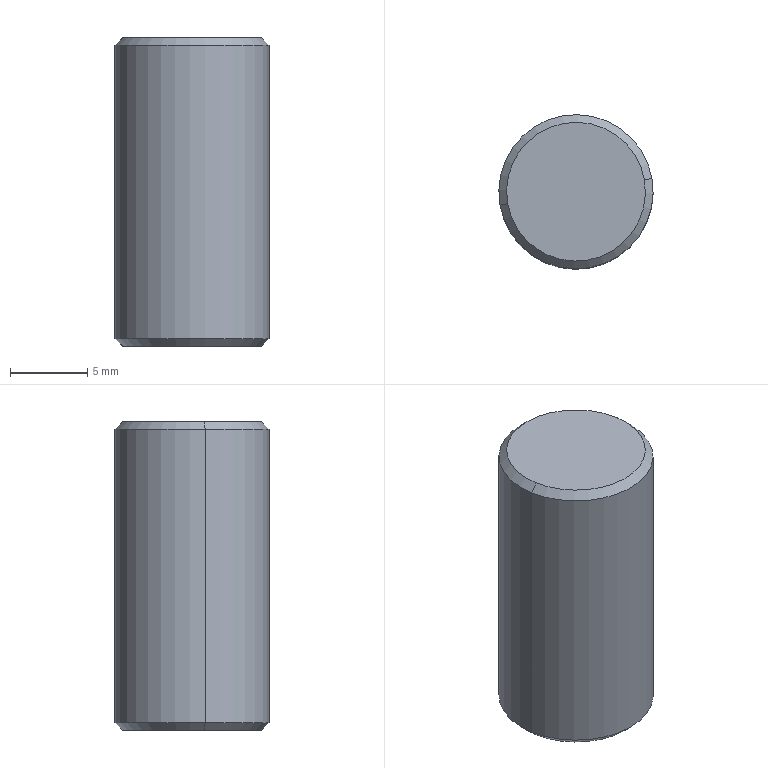Component | SolidWorks | AssemblyVibratoryFeederChassis-1_AssemblyWheel-3_WheelRetainingPin-1 | 1 solid | 8 faces | box 10 x 10 x 20 mm | volume 1563 mm3 | cone 4 | cylinder 2 | plane 2 | commonest cylinder face diameters 10 x2
build123d program:
from build123d import *

# Parameters (mm, degrees)
SKETCH2_R      = 5
EXTRUDE1_DEPTH = 20
CHAMFER1_SIZE  = 0.5


with BuildPart() as part:
    # Sketch2 → Extrude1 (new body)
    with BuildSketch(Plane.XY):
        Circle(SKETCH2_R)
    extrude(amount=EXTRUDE1_DEPTH)

    # Chamfer1
    chamfer1_edges = [part.edges().sort_by_distance(p)[0] for p in [
        (-5, 0, 0),
        (-5, 0, 20),
    ]]
    chamfer(chamfer1_edges, length=CHAMFER1_SIZE)


solid = part.part

# Placed as in the assembly
solid = solid.moved(Location((-277.449, 248.824, -92), (0, 0, 0)))
STEP:
#1=COLOUR_RGB('',0.7922,0.8196,0.9333);
#2=FILL_AREA_STYLE_COLOUR('',#1);
#3=FILL_AREA_STYLE('',(#2));
#4=SURFACE_STYLE_FILL_AREA(#3);
#5=SURFACE_SIDE_STYLE('',(#4));
#6=SURFACE_STYLE_USAGE(.BOTH.,#5);
#7=PRESENTATION_STYLE_ASSIGNMENT((#6));
#8=CARTESIAN_POINT('',(-10.749,9.827,-3.622));
#9=VERTEX_POINT('',#8);
#10=CARTESIAN_POINT('',(-11.098,9.766,-3.622));
#11=VERTEX_POINT('',#10);
#12=CARTESIAN_POINT('',(-10.923,9.796,-3.622));
#13=DIRECTION('',(-0.,-0.,-1.));
#14=DIRECTION('',(0.9851,0.1722,0.));
#15=AXIS2_PLACEMENT_3D('',#12,#13,#14);
#16=CIRCLE('',#15,0.1772);
#17=EDGE_CURVE('',#9,#11,#16,.T.);
#18=ORIENTED_EDGE('',*,*,#17,.F.);
#19=CARTESIAN_POINT('',(-10.729,9.83,-3.602));
#20=VERTEX_POINT('',#19);
#21=CARTESIAN_POINT('',(-10.749,9.827,-3.622));
#22=DIRECTION('',(0.6965,0.1217,0.7071));
#23=VECTOR('',#22,39.37);
#24=LINE('',#21,#23);
#25=EDGE_CURVE('',#9,#20,#24,.T.);
#26=ORIENTED_EDGE('',*,*,#25,.T.);
#27=CARTESIAN_POINT('',(-11.117,9.762,-3.602));
#28=VERTEX_POINT('',#27);
#29=CARTESIAN_POINT('',(-10.923,9.796,-3.602));
#30=DIRECTION('',(0.,0.,1.));
#31=DIRECTION('',(0.9851,0.1722,0.));
#32=AXIS2_PLACEMENT_3D('',#29,#30,#31);
#33=CIRCLE('',#32,0.1969);
#34=EDGE_CURVE('',#28,#20,#33,.T.);
#35=ORIENTED_EDGE('',*,*,#34,.F.);
#36=CARTESIAN_POINT('',(-11.098,9.766,-3.622));
#37=DIRECTION('',(-0.6965,-0.1217,0.7071));
#38=VECTOR('',#37,39.37);
#39=LINE('',#36,#38);
#40=EDGE_CURVE('',#11,#28,#39,.T.);
#41=ORIENTED_EDGE('',*,*,#40,.F.);
#42=EDGE_LOOP('',(#18,#26,#35,#41));
#43=FACE_OUTER_BOUND('',#42,.T.);
#44=CARTESIAN_POINT('',(-10.923,9.796,-3.622));
#45=DIRECTION('',(0.,0.,1.));
#46=DIRECTION('',(-0.9851,-0.1722,0.));
#47=AXIS2_PLACEMENT_3D('',#44,#45,#46);
#48=CONICAL_SURFACE('',#47,0.1772,0.7854);
#49=ADVANCED_FACE('',(#43),#48,.T.);
#50=CARTESIAN_POINT('',(-11.098,9.766,-2.835));
#51=VERTEX_POINT('',#50);
#52=CARTESIAN_POINT('',(-10.749,9.827,-2.835));
#53=VERTEX_POINT('',#52);
#54=CARTESIAN_POINT('',(-10.923,9.796,-2.835));
#55=DIRECTION('',(0.,0.,1.));
#56=DIRECTION('',(0.9851,0.1722,0.));
#57=AXIS2_PLACEMENT_3D('',#54,#55,#56);
#58=CIRCLE('',#57,0.1772);
#59=EDGE_CURVE('',#51,#53,#58,.T.);
#60=ORIENTED_EDGE('',*,*,#59,.F.);
#61=CARTESIAN_POINT('',(-11.117,9.762,-2.854));
#62=VERTEX_POINT('',#61);
#63=CARTESIAN_POINT('',(-11.117,9.762,-2.854));
#64=DIRECTION('',(-0.6965,-0.1217,-0.7071));
#65=VECTOR('',#64,39.37);
#66=LINE('',#63,#65);
#67=EDGE_CURVE('',#51,#62,#66,.T.);
#68=ORIENTED_EDGE('',*,*,#67,.T.);
#69=CARTESIAN_POINT('',(-10.729,9.83,-2.854));
#70=VERTEX_POINT('',#69);
#71=CARTESIAN_POINT('',(-10.923,9.796,-2.854));
#72=DIRECTION('',(-0.,-0.,-1.));
#73=DIRECTION('',(0.9851,0.1722,0.));
#74=AXIS2_PLACEMENT_3D('',#71,#72,#73);
#75=CIRCLE('',#74,0.1969);
#76=EDGE_CURVE('',#70,#62,#75,.T.);
#77=ORIENTED_EDGE('',*,*,#76,.F.);
#78=CARTESIAN_POINT('',(-10.729,9.83,-2.854));
#79=DIRECTION('',(0.6965,0.1217,-0.7071));
#80=VECTOR('',#79,39.37);
#81=LINE('',#78,#80);
#82=EDGE_CURVE('',#53,#70,#81,.T.);
#83=ORIENTED_EDGE('',*,*,#82,.F.);
#84=EDGE_LOOP('',(#60,#68,#77,#83));
#85=FACE_OUTER_BOUND('',#84,.T.);
#86=CARTESIAN_POINT('',(-10.923,9.796,-2.854));
#87=DIRECTION('',(-0.,-0.,-1.));
#88=DIRECTION('',(0.9851,0.1722,0.));
#89=AXIS2_PLACEMENT_3D('',#86,#87,#88);
#90=CONICAL_SURFACE('',#89,0.1969,0.7854);
#91=ADVANCED_FACE('',(#85),#90,.T.);
#92=ORIENTED_EDGE('',*,*,#34,.T.);
#93=CARTESIAN_POINT('',(-10.729,9.83,-3.622));
#94=DIRECTION('',(0.,0.,1.));
#95=VECTOR('',#94,39.37);
#96=LINE('',#93,#95);
#97=EDGE_CURVE('',#20,#70,#96,.T.);
#98=ORIENTED_EDGE('',*,*,#97,.T.);
#99=ORIENTED_EDGE('',*,*,#76,.T.);
#100=CARTESIAN_POINT('',(-11.117,9.762,-3.622));
#101=DIRECTION('',(0.,0.,1.));
#102=VECTOR('',#101,39.37);
#103=LINE('',#100,#102);
#104=EDGE_CURVE('',#28,#62,#103,.T.);
#105=ORIENTED_EDGE('',*,*,#104,.F.);
#106=EDGE_LOOP('',(#92,#98,#99,#105));
#107=FACE_OUTER_BOUND('',#106,.T.);
#108=CARTESIAN_POINT('',(-10.923,9.796,-3.622));
#109=DIRECTION('',(0.,0.,1.));
#110=DIRECTION('',(-0.9851,-0.1722,0.));
#111=AXIS2_PLACEMENT_3D('',#108,#109,#110);
#112=CYLINDRICAL_SURFACE('',#111,0.1969);
#113=ADVANCED_FACE('',(#107),#112,.T.);
#114=ORIENTED_EDGE('',*,*,#97,.F.);
#115=CARTESIAN_POINT('',(-10.923,9.796,-3.602));
#116=DIRECTION('',(0.,0.,1.));
#117=DIRECTION('',(0.9851,0.1722,0.));
#118=AXIS2_PLACEMENT_3D('',#115,#116,#117);
#119=CIRCLE('',#118,0.1969);
#120=EDGE_CURVE('',#20,#28,#119,.T.);
#121=ORIENTED_EDGE('',*,*,#120,.T.);
#122=ORIENTED_EDGE('',*,*,#104,.T.);
#123=CARTESIAN_POINT('',(-10.923,9.796,-2.854));
#124=DIRECTION('',(-0.,-0.,-1.));
#125=DIRECTION('',(0.9851,0.1722,0.));
#126=AXIS2_PLACEMENT_3D('',#123,#124,#125);
#127=CIRCLE('',#126,0.1969);
#128=EDGE_CURVE('',#62,#70,#127,.T.);
#129=ORIENTED_EDGE('',*,*,#128,.T.);
#130=EDGE_LOOP('',(#114,#121,#122,#129));
#131=FACE_OUTER_BOUND('',#130,.T.);
#132=CARTESIAN_POINT('',(-10.923,9.796,-3.622));
#133=DIRECTION('',(0.,0.,1.));
#134=DIRECTION('',(-0.9851,-0.1722,0.));
#135=AXIS2_PLACEMENT_3D('',#132,#133,#134);
#136=CYLINDRICAL_SURFACE('',#135,0.1969);
#137=ADVANCED_FACE('',(#131),#136,.T.);
#138=CARTESIAN_POINT('',(-10.923,9.796,-3.622));
#139=DIRECTION('',(-0.,-0.,-1.));
#140=DIRECTION('',(0.9851,0.1722,0.));
#141=AXIS2_PLACEMENT_3D('',#138,#139,#140);
#142=CIRCLE('',#141,0.1772);
#143=EDGE_CURVE('',#11,#9,#142,.T.);
#144=ORIENTED_EDGE('',*,*,#143,.T.);
#145=ORIENTED_EDGE('',*,*,#17,.T.);
#146=EDGE_LOOP('',(#144,#145));
#147=FACE_OUTER_BOUND('',#146,.T.);
#148=CARTESIAN_POINT('',(-10.923,9.796,-3.622));
#149=DIRECTION('',(-0.,-0.,-1.));
#150=DIRECTION('',(0.9851,0.1722,-0.));
#151=AXIS2_PLACEMENT_3D('',#148,#149,#150);
#152=PLANE('',#151);
#153=ADVANCED_FACE('',(#147),#152,.T.);
#154=CARTESIAN_POINT('',(-10.923,9.796,-2.835));
#155=DIRECTION('',(0.,0.,1.));
#156=DIRECTION('',(0.9851,0.1722,0.));
#157=AXIS2_PLACEMENT_3D('',#154,#155,#156);
#158=CIRCLE('',#157,0.1772);
#159=EDGE_CURVE('',#53,#51,#158,.T.);
#160=ORIENTED_EDGE('',*,*,#159,.T.);
#161=ORIENTED_EDGE('',*,*,#59,.T.);
#162=EDGE_LOOP('',(#160,#161));
#163=FACE_OUTER_BOUND('',#162,.T.);
#164=CARTESIAN_POINT('',(-10.923,9.796,-2.835));
#165=DIRECTION('',(-0.,-0.,-1.));
#166=DIRECTION('',(0.9851,0.1722,-0.));
#167=AXIS2_PLACEMENT_3D('',#164,#165,#166);
#168=PLANE('',#167);
#169=ADVANCED_FACE('',(#163),#168,.F.);
#170=ORIENTED_EDGE('',*,*,#67,.F.);
#171=ORIENTED_EDGE('',*,*,#159,.F.);
#172=ORIENTED_EDGE('',*,*,#82,.T.);
#173=ORIENTED_EDGE('',*,*,#128,.F.);
#174=EDGE_LOOP('',(#170,#171,#172,#173));
#175=FACE_OUTER_BOUND('',#174,.T.);
#176=CARTESIAN_POINT('',(-10.923,9.796,-2.854));
#177=DIRECTION('',(-0.,-0.,-1.));
#178=DIRECTION('',(0.9851,0.1722,0.));
#179=AXIS2_PLACEMENT_3D('',#176,#177,#178);
#180=CONICAL_SURFACE('',#179,0.1969,0.7854);
#181=ADVANCED_FACE('',(#175),#180,.T.);
#182=ORIENTED_EDGE('',*,*,#25,.F.);
#183=ORIENTED_EDGE('',*,*,#143,.F.);
#184=ORIENTED_EDGE('',*,*,#40,.T.);
#185=ORIENTED_EDGE('',*,*,#120,.F.);
#186=EDGE_LOOP('',(#182,#183,#184,#185));
#187=FACE_OUTER_BOUND('',#186,.T.);
#188=CARTESIAN_POINT('',(-10.923,9.796,-3.622));
#189=DIRECTION('',(0.,0.,1.));
#190=DIRECTION('',(-0.9851,-0.1722,0.));
#191=AXIS2_PLACEMENT_3D('',#188,#189,#190);
#192=CONICAL_SURFACE('',#191,0.1772,0.7854);
#193=ADVANCED_FACE('',(#187),#192,.T.);
#194=CLOSED_SHELL('',(#49,#91,#113,#137,#153,#169,#181,#193));
#195=MANIFOLD_SOLID_BREP('',#194);
#196=STYLED_ITEM('',(#7),#195);
#197=PRESENTATION_LAYER_ASSIGNMENT('','',(#196));
#198=CARTESIAN_POINT('',(0.,0.,0.));
#199=DIRECTION('',(0.,0.,1.));
#200=DIRECTION('',(1.,0.,0.));
#201=AXIS2_PLACEMENT_3D('',#198,#199,#200);
#202=(LENGTH_UNIT()NAMED_UNIT(*)SI_UNIT($,.METRE.));
#203=LENGTH_MEASURE_WITH_UNIT(LENGTH_MEASURE(0.0254),#202);
#204=DIMENSIONAL_EXPONENTS(1.,0.,0.,0.,0.,0.,0.);
#205=(CONVERSION_BASED_UNIT('',#203)LENGTH_UNIT()NAMED_UNIT(#204));
#206=UNCERTAINTY_MEASURE_WITH_UNIT(LENGTH_MEASURE(0.00001),#205,'','');
#207=(NAMED_UNIT(*)PLANE_ANGLE_UNIT()SI_UNIT($,.RADIAN.));
#208=(NAMED_UNIT(*)SI_UNIT($,.STERADIAN.)SOLID_ANGLE_UNIT());
#209=(GEOMETRIC_REPRESENTATION_CONTEXT(3)GLOBAL_UNCERTAINTY_ASSIGNED_CONTEXT((#206))GLOBAL_UNIT_ASSIGNED_CONTEXT((#205,#207,#208))REPRESENTATION_CONTEXT('',''));
#210=ADVANCED_BREP_SHAPE_REPRESENTATION('',(#195,#201),#209);
#211=(LENGTH_UNIT()NAMED_UNIT(*)SI_UNIT($,.METRE.));
#212=LENGTH_MEASURE_WITH_UNIT(LENGTH_MEASURE(0.0254),#211);
#213=DIMENSIONAL_EXPONENTS(1.,0.,0.,0.,0.,0.,0.);
#214=(CONVERSION_BASED_UNIT('',#212)LENGTH_UNIT()NAMED_UNIT(#213));
#215=UNCERTAINTY_MEASURE_WITH_UNIT(LENGTH_MEASURE(0.00001),#214,'','');
#216=(NAMED_UNIT(*)PLANE_ANGLE_UNIT()SI_UNIT($,.RADIAN.));
#217=(NAMED_UNIT(*)SI_UNIT($,.STERADIAN.)SOLID_ANGLE_UNIT());
#218=(GEOMETRIC_REPRESENTATION_CONTEXT(3)GLOBAL_UNCERTAINTY_ASSIGNED_CONTEXT((#215))GLOBAL_UNIT_ASSIGNED_CONTEXT((#214,#216,#217))REPRESENTATION_CONTEXT('',''));
#219=MECHANICAL_DESIGN_GEOMETRIC_PRESENTATION_REPRESENTATION('',(#196),#218);